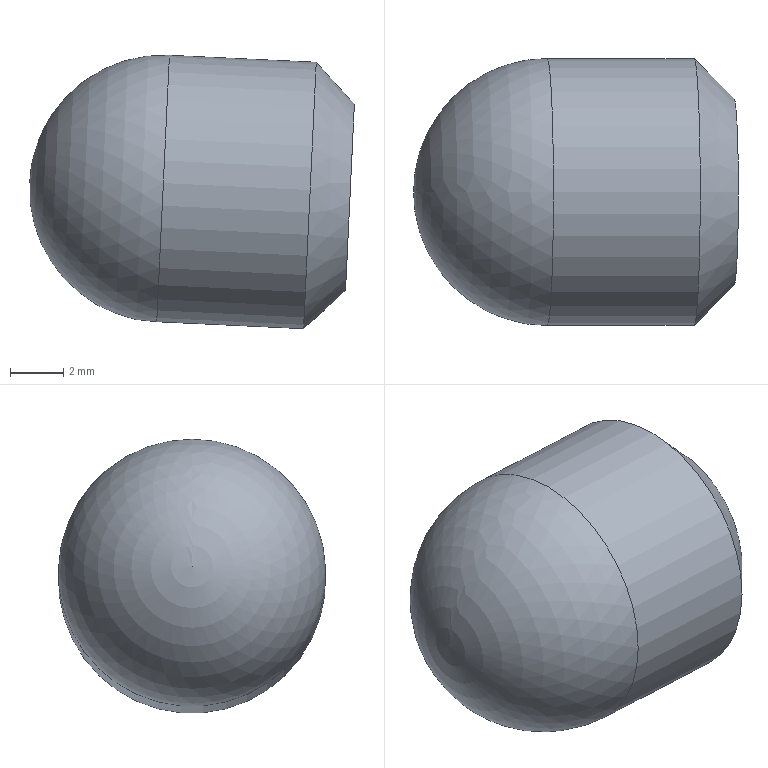Component | NX | LIQUID_COLUMN | 1 solid | 4 faces | box 12.16 x 10 x 10.26 mm | volume 780 mm3 | plane 1 | cylinder 1 | sphere 1 | cone 1 | commonest cylinder face diameters 10 x1
STEP:
#1=CARTESIAN_POINT('',(0.,0.,0.));
#2=DIRECTION('',(0.,0.,1.));
#3=DIRECTION('',(1.,0.,0.));
#4=AXIS2_PLACEMENT_3D('',#1,#2,#3);
#5=CARTESIAN_POINT('',(-2.63,-52.911,2.681));
#6=VERTEX_POINT('',#5);
#7=CARTESIAN_POINT('',(-2.796,-52.911,-0.815));
#8=DIRECTION('',(0.9989,0.,-0.04757));
#9=DIRECTION('',(0.04757,0.,0.9989));
#10=AXIS2_PLACEMENT_3D('',#7,#8,#9);
#11=CIRCLE('',#10,3.5);
#12=CARTESIAN_POINT('',(-2.796,-52.911,-0.815));
#13=DIRECTION('',(-0.9989,0.,0.04757));
#14=DIRECTION('',(0.04757,0.,0.9989));
#15=AXIS2_PLACEMENT_3D('',#12,#13,#14);
#16=PLANE('',#15);
#17=CARTESIAN_POINT('',(3.5,0.));
#18=CARTESIAN_POINT('',(3.5,-6.062));
#19=CARTESIAN_POINT('',(-1.75,-3.031));
#20=CARTESIAN_POINT('',(-7.,-0.));
#21=CARTESIAN_POINT('',(-1.75,3.031));
#22=CARTESIAN_POINT('',(3.5,6.062));
#23=CARTESIAN_POINT('',(3.5,0.));
#24=(BOUNDED_CURVE()B_SPLINE_CURVE(2,(#17,#18,#19,#20,#21,#22,#23),.UNSPECIFIED.,.T.,.F.)B_SPLINE_CURVE_WITH_KNOTS((1,2,2,2,2,1),(-2.094,0.,2.094,4.189,6.283,8.378),.UNSPECIFIED.)CURVE()GEOMETRIC_REPRESENTATION_ITEM()RATIONAL_B_SPLINE_CURVE((1.,0.5,1.,0.5,1.,0.5,1.))REPRESENTATION_ITEM(''));
#25=(GEOMETRIC_REPRESENTATION_CONTEXT(2)PARAMETRIC_REPRESENTATION_CONTEXT()REPRESENTATION_CONTEXT('',''));
#26=DEFINITIONAL_REPRESENTATION('',(#24),#25);
#27=PCURVE('',#16,#26);
#28=CARTESIAN_POINT('',(-4.295,-52.911,-0.7437));
#29=DIRECTION('',(-0.9989,0.,0.04757));
#30=DIRECTION('',(0.04757,0.,0.9989));
#31=AXIS2_PLACEMENT_3D('',#28,#29,#30);
#32=CONICAL_SURFACE('',#31,5.,0.7854);
#33=CARTESIAN_POINT('',(6.283,-1.5));
#34=DIRECTION('',(-1.,0.));
#35=VECTOR('',#34,1.);
#36=LINE('',#33,#35);
#37=(GEOMETRIC_REPRESENTATION_CONTEXT(2)PARAMETRIC_REPRESENTATION_CONTEXT()REPRESENTATION_CONTEXT('',''));
#38=DEFINITIONAL_REPRESENTATION('',(#36),#37);
#39=PCURVE('',#32,#38);
#40=SURFACE_CURVE('',#11,(#27,#39),.PCURVE_S1.);
#41=EDGE_CURVE('',#6,#6,#40,.T.);
#42=ORIENTED_EDGE('',*,*,#41,.T.);
#43=EDGE_LOOP('',(#42));
#44=FACE_BOUND('',#43,.T.);
#45=ADVANCED_FACE('',(#44),#16,.F.);
#46=CARTESIAN_POINT('',(-4.057,-52.911,4.251));
#47=VERTEX_POINT('',#46);
#48=CARTESIAN_POINT('',(-4.295,-52.911,-0.7437));
#49=DIRECTION('',(-0.9989,0.,0.04757));
#50=DIRECTION('',(0.04757,0.,0.9989));
#51=AXIS2_PLACEMENT_3D('',#48,#49,#50);
#52=CIRCLE('',#51,5.);
#53=CARTESIAN_POINT('',(-2.796,-52.911,-0.815));
#54=DIRECTION('',(-0.9989,0.,0.04757));
#55=DIRECTION('',(0.04757,0.,0.9989));
#56=AXIS2_PLACEMENT_3D('',#53,#54,#55);
#57=CYLINDRICAL_SURFACE('',#56,5.);
#58=CARTESIAN_POINT('',(0.,1.5));
#59=DIRECTION('',(1.,0.));
#60=VECTOR('',#59,1.);
#61=LINE('',#58,#60);
#62=(GEOMETRIC_REPRESENTATION_CONTEXT(2)PARAMETRIC_REPRESENTATION_CONTEXT()REPRESENTATION_CONTEXT('',''));
#63=DEFINITIONAL_REPRESENTATION('',(#61),#62);
#64=PCURVE('',#57,#63);
#65=CARTESIAN_POINT('',(0.,0.));
#66=DIRECTION('',(1.,0.));
#67=VECTOR('',#66,1.);
#68=LINE('',#65,#67);
#69=(GEOMETRIC_REPRESENTATION_CONTEXT(2)PARAMETRIC_REPRESENTATION_CONTEXT()REPRESENTATION_CONTEXT('',''));
#70=DEFINITIONAL_REPRESENTATION('',(#68),#69);
#71=PCURVE('',#32,#70);
#72=SURFACE_CURVE('',#52,(#64,#71),.PCURVE_S1.);
#73=EDGE_CURVE('',#47,#47,#72,.T.);
#74=ORIENTED_EDGE('',*,*,#73,.T.);
#75=CARTESIAN_POINT('',(-9.551,-52.911,4.512));
#76=VERTEX_POINT('',#75);
#77=CARTESIAN_POINT('',(-4.057,-52.911,4.251));
#78=CARTESIAN_POINT('',(-9.551,-52.911,4.512));
#79=B_SPLINE_CURVE_WITH_KNOTS('',1,(#77,#78),.UNSPECIFIED.,.F.,.F.,(2,2),(1.5,7.),.PIECEWISE_BEZIER_KNOTS.);
#80=CARTESIAN_POINT('',(6.283,0.));
#81=DIRECTION('',(0.,1.));
#82=VECTOR('',#81,1.);
#83=LINE('',#80,#82);
#84=(GEOMETRIC_REPRESENTATION_CONTEXT(2)PARAMETRIC_REPRESENTATION_CONTEXT()REPRESENTATION_CONTEXT('',''));
#85=DEFINITIONAL_REPRESENTATION('',(#83),#84);
#86=PCURVE('',#57,#85);
#87=CARTESIAN_POINT('',(0.,0.));
#88=DIRECTION('',(0.,1.));
#89=VECTOR('',#88,1.);
#90=LINE('',#87,#89);
#91=(GEOMETRIC_REPRESENTATION_CONTEXT(2)PARAMETRIC_REPRESENTATION_CONTEXT()REPRESENTATION_CONTEXT('',''));
#92=DEFINITIONAL_REPRESENTATION('',(#90),#91);
#93=PCURVE('',#57,#92);
#94=SEAM_CURVE('',#79,(#86,#93),.PCURVE_S1.);
#95=EDGE_CURVE('',#47,#76,#94,.T.);
#96=ORIENTED_EDGE('',*,*,#95,.T.);
#97=CARTESIAN_POINT('',(-9.789,-52.911,-0.4821));
#98=DIRECTION('',(-0.9989,0.,0.04757));
#99=DIRECTION('',(0.04757,0.,0.9989));
#100=AXIS2_PLACEMENT_3D('',#97,#98,#99);
#101=CIRCLE('',#100,5.);
#102=CARTESIAN_POINT('',(0.,7.));
#103=DIRECTION('',(1.,0.));
#104=VECTOR('',#103,1.);
#105=LINE('',#102,#104);
#106=(GEOMETRIC_REPRESENTATION_CONTEXT(2)PARAMETRIC_REPRESENTATION_CONTEXT()REPRESENTATION_CONTEXT('',''));
#107=DEFINITIONAL_REPRESENTATION('',(#105),#106);
#108=PCURVE('',#57,#107);
#109=CARTESIAN_POINT('',(-9.789,-52.911,-0.4821));
#110=DIRECTION('',(-0.9989,0.,0.04757));
#111=DIRECTION('',(0.04757,0.,0.9989));
#112=AXIS2_PLACEMENT_3D('',#109,#110,#111);
#113=SPHERICAL_SURFACE('',#112,5.);
#114=CARTESIAN_POINT('',(0.,-0.));
#115=CARTESIAN_POINT('',(0.0952,-0.));
#116=CARTESIAN_POINT('',(0.2856,0.));
#117=CARTESIAN_POINT('',(0.5712,-0.));
#118=CARTESIAN_POINT('',(0.8568,0.));
#119=CARTESIAN_POINT('',(1.142,-0.));
#120=CARTESIAN_POINT('',(1.428,0.));
#121=CARTESIAN_POINT('',(1.714,-0.));
#122=CARTESIAN_POINT('',(1.999,-0.));
#123=CARTESIAN_POINT('',(2.285,-0.));
#124=CARTESIAN_POINT('',(2.57,0.));
#125=CARTESIAN_POINT('',(2.856,-0.));
#126=CARTESIAN_POINT('',(3.142,0.));
#127=CARTESIAN_POINT('',(3.427,-0.));
#128=CARTESIAN_POINT('',(3.713,0.));
#129=CARTESIAN_POINT('',(3.998,-0.));
#130=CARTESIAN_POINT('',(4.284,-0.));
#131=CARTESIAN_POINT('',(4.57,-0.));
#132=CARTESIAN_POINT('',(4.855,0.));
#133=CARTESIAN_POINT('',(5.141,-0.));
#134=CARTESIAN_POINT('',(5.426,0.));
#135=CARTESIAN_POINT('',(5.712,-0.));
#136=CARTESIAN_POINT('',(5.998,0.));
#137=CARTESIAN_POINT('',(6.188,-0.));
#138=CARTESIAN_POINT('',(6.283,-0.));
#139=B_SPLINE_CURVE_WITH_KNOTS('',3,(#114,#115,#116,#117,#118,#119,#120,#121,#122,#123,#124,#125,#126,#127,#128,#129,#130,#131,#132,#133,#134,#135,#136,#137,#138),.UNSPECIFIED.,.F.,.F.,(4,1,1,1,1,1,1,1,1,1,1,1,1,1,1,1,1,1,1,1,1,1,4),(0.,0.2856,0.5712,0.8568,1.142,1.428,1.714,1.999,2.285,2.57,2.856,3.142,3.427,3.713,3.998,4.284,4.57,4.855,5.141,5.426,5.712,5.998,6.283),.QUASI_UNIFORM_KNOTS.);
#140=(GEOMETRIC_REPRESENTATION_CONTEXT(2)PARAMETRIC_REPRESENTATION_CONTEXT()REPRESENTATION_CONTEXT('',''));
#141=DEFINITIONAL_REPRESENTATION('',(#139),#140);
#142=PCURVE('',#113,#141);
#143=SURFACE_CURVE('',#101,(#108,#142),.PCURVE_S1.);
#144=EDGE_CURVE('',#76,#76,#143,.T.);
#145=ORIENTED_EDGE('',*,*,#144,.F.);
#146=ORIENTED_EDGE('',*,*,#95,.F.);
#147=EDGE_LOOP('',(#74,#96,#145,#146));
#148=FACE_BOUND('',#147,.T.);
#149=ADVANCED_FACE('',(#148),#57,.T.);
#150=ORIENTED_EDGE('',*,*,#144,.T.);
#151=CARTESIAN_POINT('',(-14.783,-52.911,-0.2442));
#152=VERTEX_POINT('',#151);
#153=CARTESIAN_POINT('',(-9.551,-52.911,4.512));
#154=CARTESIAN_POINT('',(-10.858,-52.911,4.575));
#155=CARTESIAN_POINT('',(-12.185,-52.911,4.226));
#156=CARTESIAN_POINT('',(-13.371,-52.911,3.459));
#157=CARTESIAN_POINT('',(-14.248,-52.911,2.351));
#158=CARTESIAN_POINT('',(-14.721,-52.911,1.063));
#159=CARTESIAN_POINT('',(-14.783,-52.911,-0.2442));
#160=B_SPLINE_CURVE_WITH_KNOTS('',6,(#153,#154,#155,#156,#157,#158,#159),.UNSPECIFIED.,.F.,.F.,(7,7),(-0.,1.571),.PIECEWISE_BEZIER_KNOTS.);
#161=CARTESIAN_POINT('',(6.283,0.));
#162=DIRECTION('',(0.,1.));
#163=VECTOR('',#162,1.);
#164=LINE('',#161,#163);
#165=(GEOMETRIC_REPRESENTATION_CONTEXT(2)PARAMETRIC_REPRESENTATION_CONTEXT()REPRESENTATION_CONTEXT('',''));
#166=DEFINITIONAL_REPRESENTATION('',(#164),#165);
#167=PCURVE('',#113,#166);
#168=CARTESIAN_POINT('',(0.,0.));
#169=DIRECTION('',(0.,1.));
#170=VECTOR('',#169,1.);
#171=LINE('',#168,#170);
#172=(GEOMETRIC_REPRESENTATION_CONTEXT(2)PARAMETRIC_REPRESENTATION_CONTEXT()REPRESENTATION_CONTEXT('',''));
#173=DEFINITIONAL_REPRESENTATION('',(#171),#172);
#174=PCURVE('',#113,#173);
#175=SEAM_CURVE('',#160,(#167,#174),.PCURVE_S1.);
#176=EDGE_CURVE('',#76,#152,#175,.T.);
#177=ORIENTED_EDGE('',*,*,#176,.T.);
#178=ORIENTED_EDGE('',*,*,#176,.F.);
#179=EDGE_LOOP('',(#150,#177,#178));
#180=FACE_BOUND('',#179,.T.);
#181=ADVANCED_FACE('',(#180),#113,.T.);
#182=ORIENTED_EDGE('',*,*,#41,.F.);
#183=CARTESIAN_POINT('',(-2.63,-52.911,2.681));
#184=CARTESIAN_POINT('',(-4.057,-52.911,4.251));
#185=B_SPLINE_CURVE_WITH_KNOTS('',1,(#183,#184),.UNSPECIFIED.,.F.,.F.,(2,2),(-2.121,0.),.PIECEWISE_BEZIER_KNOTS.);
#186=CARTESIAN_POINT('',(6.283,0.));
#187=DIRECTION('',(0.,1.));
#188=VECTOR('',#187,1.);
#189=LINE('',#186,#188);
#190=(GEOMETRIC_REPRESENTATION_CONTEXT(2)PARAMETRIC_REPRESENTATION_CONTEXT()REPRESENTATION_CONTEXT('',''));
#191=DEFINITIONAL_REPRESENTATION('',(#189),#190);
#192=PCURVE('',#32,#191);
#193=CARTESIAN_POINT('',(0.,0.));
#194=DIRECTION('',(0.,1.));
#195=VECTOR('',#194,1.);
#196=LINE('',#193,#195);
#197=(GEOMETRIC_REPRESENTATION_CONTEXT(2)PARAMETRIC_REPRESENTATION_CONTEXT()REPRESENTATION_CONTEXT('',''));
#198=DEFINITIONAL_REPRESENTATION('',(#196),#197);
#199=PCURVE('',#32,#198);
#200=SEAM_CURVE('',#185,(#192,#199),.PCURVE_S1.);
#201=EDGE_CURVE('',#6,#47,#200,.T.);
#202=ORIENTED_EDGE('',*,*,#201,.T.);
#203=ORIENTED_EDGE('',*,*,#73,.F.);
#204=ORIENTED_EDGE('',*,*,#201,.F.);
#205=EDGE_LOOP('',(#182,#202,#203,#204));
#206=FACE_BOUND('',#205,.T.);
#207=ADVANCED_FACE('',(#206),#32,.T.);
#208=CLOSED_SHELL('',(#45,#149,#181,#207));
#209=MANIFOLD_SOLID_BREP('',#208);
#210=(LENGTH_UNIT()NAMED_UNIT(*)SI_UNIT(.MILLI.,.METRE.));
#211=UNCERTAINTY_MEASURE_WITH_UNIT(LENGTH_MEASURE(0.00001),#210,'','');
#212=(NAMED_UNIT(*)PLANE_ANGLE_UNIT()SI_UNIT($,.RADIAN.));
#213=(NAMED_UNIT(*)SI_UNIT($,.STERADIAN.)SOLID_ANGLE_UNIT());
#214=(GEOMETRIC_REPRESENTATION_CONTEXT(3)GLOBAL_UNCERTAINTY_ASSIGNED_CONTEXT((#211))GLOBAL_UNIT_ASSIGNED_CONTEXT((#210,#212,#213))REPRESENTATION_CONTEXT('',''));
#215=ADVANCED_BREP_SHAPE_REPRESENTATION('',(#4,#209),#214);